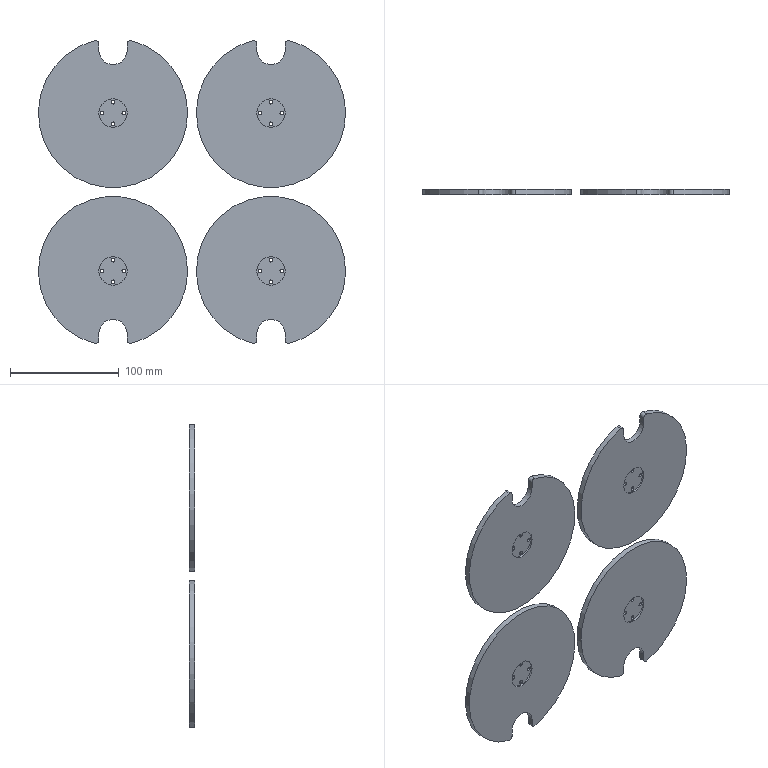CAM job | Mastercam | mm | 6 operations | part box 282 x 5 x 278.03
1. Contour (Ramp) | 3 - 3 平铣刀
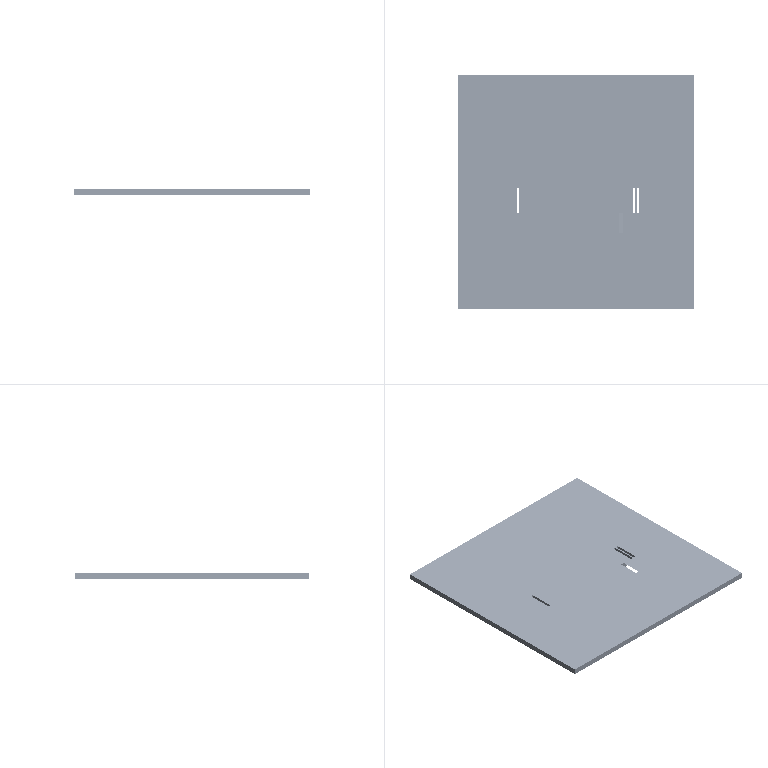2. 2D High Speed (2D Area Mill) | 3 - 3 平铣刀
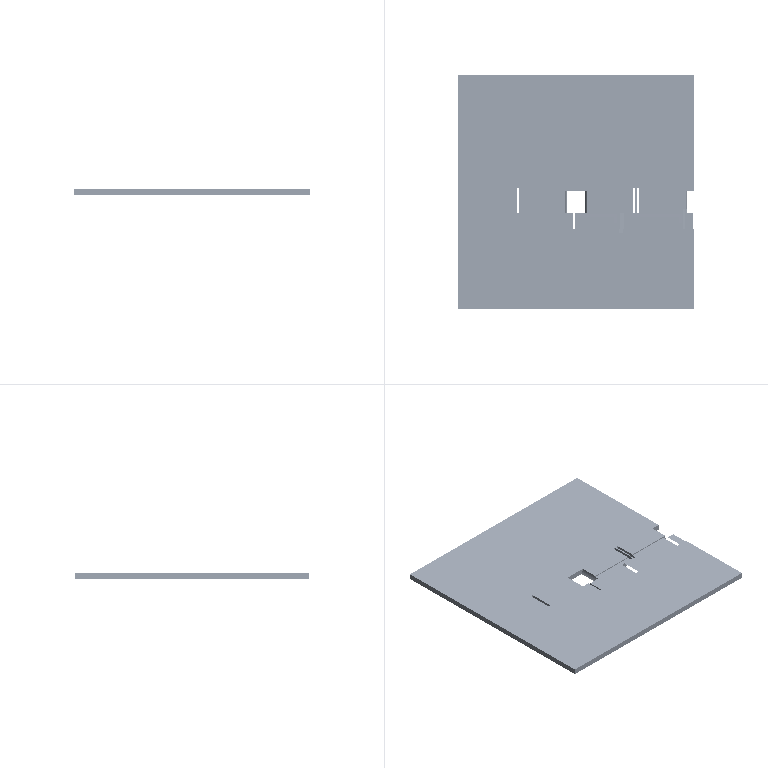3. 2D High Speed (2D Area Mill) | 3 - 3 平铣刀
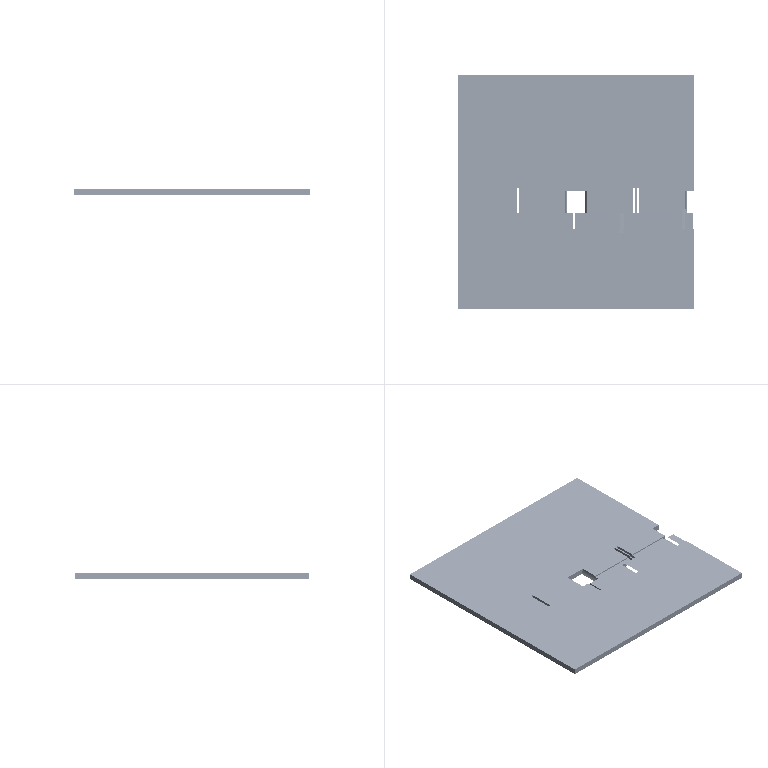4. Contour (2D chamfer) | 7 - 4 倒角刀
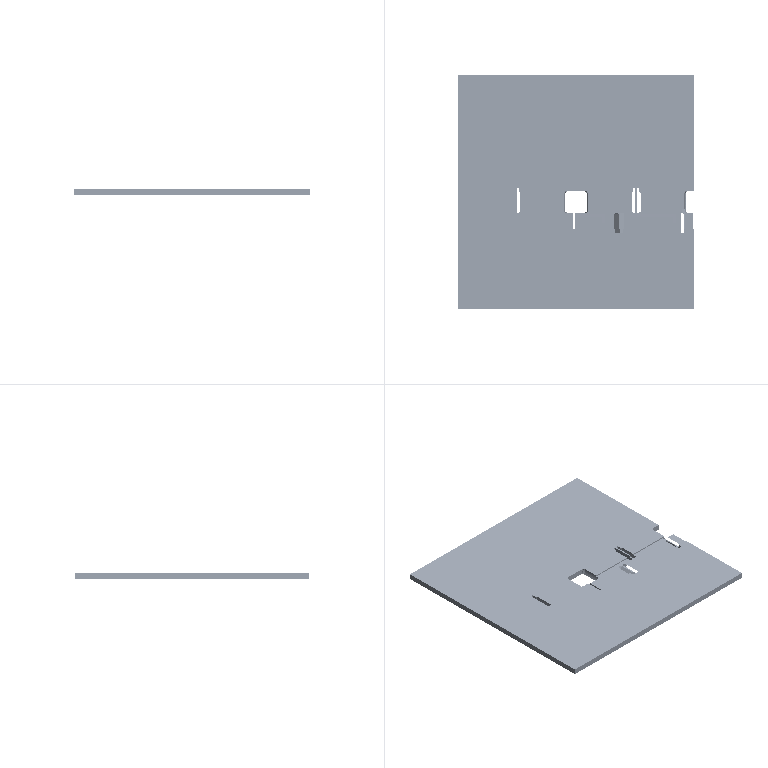5. Drill/Counterbore | 7 - 4 倒角刀
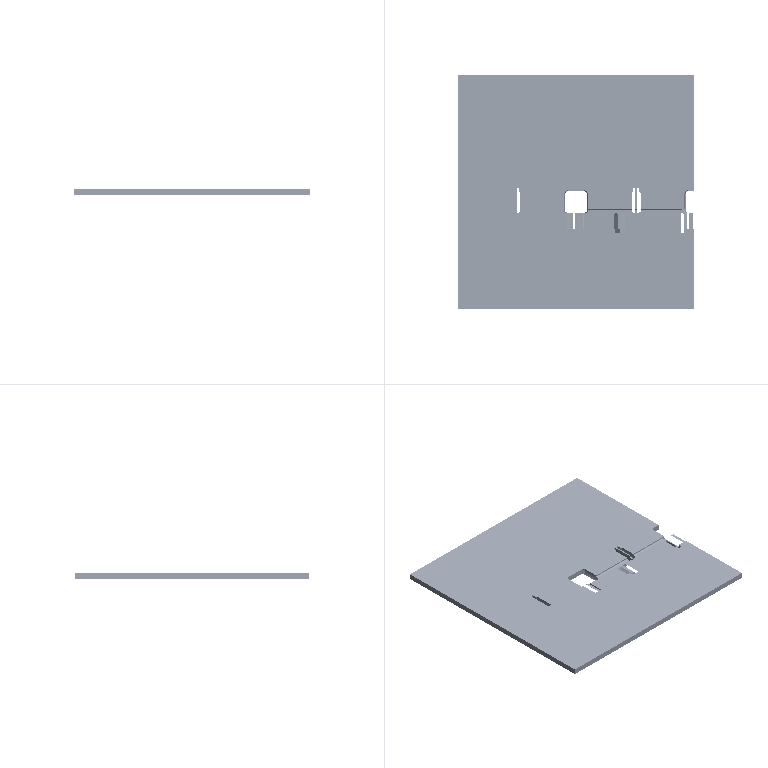6. Contour (Ramp) | 2 - 2 平铣刀